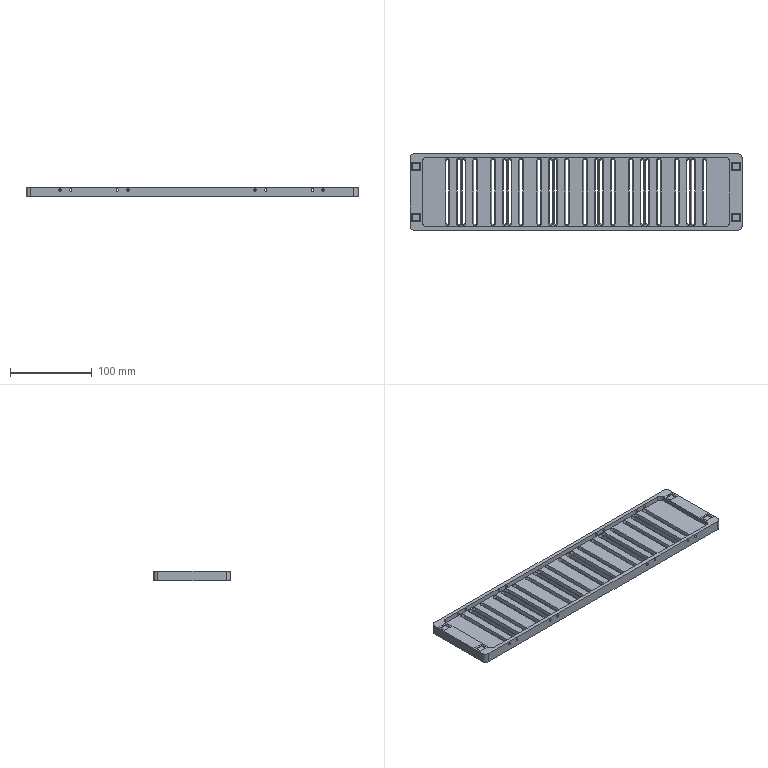Component | SolidWorks | MGL-PACK-01-00WeldedPlate1Assembly-1_MGL-PACK-01-01WeldPlate1-1 | 1 solid | 279 faces | box 405 x 93 x 12 mm | volume 214610 mm3 | plane 143 | cylinder 88 | cone 48 | commonest cylinder face diameters 3.5 x48 3 x32 10 x8
build123d program:
from build123d import *

# Parameters (mm, degrees)
SKETCH1_W             = 405
SKETCH1_H             = 93
BOSS_EXTRUDE1_DEPTH   = 12
CUT_EXTRUDE1_DEPTH    = 12
CUT_EXTRUDE4_DEPTH    = 12
LPATTERN1_COUNT       = 5
LPATTERN1_PITCH       = 56
CUT_EXTRUDE2_DEPTH    = 6
FILLET1_R             = 5
M3_TAPPED_HOLE1_D     = 3
M3_TAPPED_HOLE1_DEPTH = 120
M3_TAPPED_HOLE1_TIP   = 0.9013
SKETCH6_W             = 9
SKETCH6_H             = 8
CUT_EXTRUDE3_DEPTH    = 2
CHAMFER3_SIZE         = 1
CHAMFER4_SIZE         = 1
CHAMFER4_SIZE2        = 3.732


with BuildPart() as part:
    # Sketch1 → Boss-Extrude1 (new body)
    with BuildSketch(Plane.XY):
        Rectangle(SKETCH1_W, SKETCH1_H)
    extrude(amount=BOSS_EXTRUDE1_DEPTH)

    # Sketch2 → Cut-Extrude1 (cut)
    with BuildSketch(Plane.XY.offset(12)):
        with BuildLine():
            Line((-155.25, 38), (-155.25, -38))
            ThreePointArc((-155.25, -38), (-157, -39.75), (-158.75, -38))
            Line((-158.75, -38), (-158.75, 38))
            ThreePointArc((-158.75, 38), (-157, 39.75), (-155.25, 38))
        make_face()
        with BuildLine():
            Line((158.75, 38), (158.75, -38))
            ThreePointArc((158.75, -38), (157, -39.75), (155.25, -38))
            Line((155.25, -38), (155.25, 38))
            ThreePointArc((155.25, 38), (157, 39.75), (158.75, 38))
        make_face()
        with BuildLine():
            Line((-141.25, 38), (-141.25, -38))
            ThreePointArc((-141.25, -38), (-143, -39.75), (-144.75, -38))
            Line((-144.75, -38), (-144.75, 38))
            ThreePointArc((-144.75, 38), (-143, 39.75), (-141.25, 38))
        make_face()
        with BuildLine():
            Line((144.75, 38), (144.75, -38))
            ThreePointArc((144.75, -38), (143, -39.75), (141.25, -38))
            Line((141.25, -38), (141.25, 38))
            ThreePointArc((141.25, 38), (143, 39.75), (144.75, 38))
        make_face()
    extrude(amount=-CUT_EXTRUDE1_DEPTH, mode=Mode.SUBTRACT)

    # Sketch8 → Cut-Extrude4 (cut)
    with BuildSketch(Plane.XY.offset(12)):
        with BuildLine():
            Line((-135.25, 38), (-135.25, -38))
            ThreePointArc((-135.25, -38), (-137, -39.75), (-138.75, -38))
            Line((-138.75, -38), (-138.75, 38))
            ThreePointArc((-138.75, 38), (-137, 39.75), (-135.25, 38))
        make_face()
        with BuildLine():
            Line((-121.25, 38), (-121.25, -38))
            ThreePointArc((-121.25, -38), (-123, -39.75), (-124.75, -38))
            Line((-124.75, -38), (-124.75, 38))
            ThreePointArc((-124.75, 38), (-123, 39.75), (-121.25, 38))
        make_face()
        with BuildLine():
            Line((-99.25, 38), (-99.25, -38))
            ThreePointArc((-99.25, -38), (-101, -39.75), (-102.75, -38))
            Line((-102.75, -38), (-102.75, 38))
            ThreePointArc((-102.75, 38), (-101, 39.75), (-99.25, 38))
        make_face()
        with BuildLine():
            Line((-85.25, 38), (-85.25, -38))
            ThreePointArc((-85.25, -38), (-87, -39.75), (-88.75, -38))
            Line((-88.75, -38), (-88.75, 38))
            ThreePointArc((-88.75, 38), (-87, 39.75), (-85.25, 38))
        make_face()
    cut_extrude4 = extrude(amount=-CUT_EXTRUDE4_DEPTH, mode=Mode.SUBTRACT)

    # LPattern1: Cut-Extrude4 ×5
    with Locations(*[(i * LPATTERN1_PITCH, 0, 0) for i in range(1, LPATTERN1_COUNT)]):
        add(cut_extrude4, mode=Mode.SUBTRACT)

    # Sketch3 → Cut-Extrude2 (cut)
    with BuildSketch(Plane.XY.offset(12)):
        with BuildLine():
            Line((-182.5, 42), (182.5, 42))
            ThreePointArc((182.5, 42), (186.036, 40.536), (187.5, 37))
            Line((187.5, 37), (187.5, -37))
            ThreePointArc((187.5, -37), (186.036, -40.536), (182.5, -42))
            Line((182.5, -42), (-182.5, -42))
            ThreePointArc((-182.5, -42), (-186.036, -40.536), (-187.5, -37))
            Line((-187.5, -37), (-187.5, 37))
            ThreePointArc((-187.5, 37), (-186.036, 40.536), (-182.5, 42))
        make_face()
    extrude(amount=-CUT_EXTRUDE2_DEPTH, mode=Mode.SUBTRACT)

    # Fillet1
    fillet1_edges = [part.edges().sort_by_distance(p)[0] for p in [
        (-202.5, 46.5, 6),
        (202.5, 46.5, 6),
        (202.5, -46.5, 6),
        (-202.5, -46.5, 6),
    ]]
    fillet(fillet1_edges, radius=FILLET1_R)

    # M3 Tapped Hole1
    with Locations(Plane(origin=(0, 46.5, 0), x_dir=(1, 0, 0), z_dir=(0, 1, 0))):
        with Locations((-161.05, -8.5), (-148.05, -8.5), (146.95, -8.5), (159.95, -8.5), (-91.05, -8.5), (-78.05, -8.5), (76.95, -8.5), (89.95, -8.5)):
            Hole(M3_TAPPED_HOLE1_D / 2, depth=M3_TAPPED_HOLE1_DEPTH)
            with Locations((0, 0, -(M3_TAPPED_HOLE1_DEPTH + M3_TAPPED_HOLE1_TIP / 2))):  # 118° drill point
                Cone(0, M3_TAPPED_HOLE1_D / 2, M3_TAPPED_HOLE1_TIP, mode=Mode.SUBTRACT)

    # Sketch6 → Cut-Extrude3 (cut)
    with BuildSketch(Plane.XY.offset(12)):
        with Locations((195, 31)):
            Rectangle(SKETCH6_W, SKETCH6_H)
        with Locations((195, -31)):
            Rectangle(SKETCH6_W, SKETCH6_H)
        with Locations((-195, 31)):
            Rectangle(SKETCH6_W, SKETCH6_H)
        with Locations((-195, -31)):
            Rectangle(SKETCH6_W, SKETCH6_H)
    extrude(amount=-CUT_EXTRUDE3_DEPTH, mode=Mode.SUBTRACT)

    # Chamfer3
    chamfer3_edges = [part.edges().sort_by_distance(p)[0] for p in [
        (190.5, 31, 12),
        (195, 27, 12),
        (199.5, 31, 12),
        (195, 35, 12),
        (190.5, -31, 12),
        (195, -35, 12),
        (199.5, -31, 12),
        (195, -27, 12),
        (-199.5, 31, 12),
        (-195, 27, 12),
        (-190.5, 31, 12),
        (-195, 35, 12),
        (-199.5, -31, 12),
        (-195, -35, 12),
        (-190.5, -31, 12),
        (-195, -27, 12),
    ]]
    chamfer(chamfer3_edges, length=CHAMFER3_SIZE)

    # Chamfer4
    chamfer4_edges = [part.edges().sort_by_distance(p)[0] for p in [
        (137, 39.75, 6),
        (135.25, 0, 6),
        (137, -39.75, 6),
        (138.75, 0, 6),
        (87, 39.75, 6),
        (85.25, 0, 6),
        (87, -39.75, 6),
        (88.75, 0, 6),
        (101, 39.75, 6),
        (99.25, 0, 6),
        (101, -39.75, 6),
        (102.75, 0, 6),
        (123, 39.75, 6),
        (121.25, 0, 6),
        (123, -39.75, 6),
        (124.75, 0, 6),
        (81, 39.75, 6),
        (79.25, 0, 6),
        (81, -39.75, 6),
        (82.75, 0, 6),
        (31, 39.75, 6),
        (29.25, 0, 6),
        (31, -39.75, 6),
        (32.75, 0, 6),
        (45, 39.75, 6),
        (43.25, 0, 6),
        (45, -39.75, 6),
        (46.75, 0, 6),
        (67, 39.75, 6),
        (65.25, 0, 6),
        (67, -39.75, 6),
        (68.75, 0, 6),
        (25, 39.75, 6),
        (23.25, 0, 6),
        (25, -39.75, 6),
        (26.75, 0, 6),
        (-25, 39.75, 6),
        (-26.75, 0, 6),
        (-25, -39.75, 6),
        (-23.25, 0, 6),
        (-11, 39.75, 6),
        (-12.75, 0, 6),
        (-11, -39.75, 6),
        (-9.25, 0, 6),
        (11, 39.75, 6),
        (9.25, 0, 6),
        (11, -39.75, 6),
        (12.75, 0, 6),
        (-29.25, 0, 6),
        (-31, 39.75, 6),
        (-32.75, 0, 6),
        (-31, -39.75, 6),
        (-79.25, 0, 6),
        (-81, 39.75, 6),
        (-82.75, 0, 6),
        (-81, -39.75, 6),
        (-65.25, 0, 6),
        (-67, 39.75, 6),
        (-68.75, 0, 6),
        (-67, -39.75, 6),
        (-43.25, 0, 6),
        (-45, 39.75, 6),
        (-46.75, 0, 6),
        (-45, -39.75, 6),
        (-85.25, 0, 6),
        (-87, 39.75, 6),
        (-88.75, 0, 6),
        (-87, -39.75, 6),
        (-99.25, 0, 6),
        (-101, 39.75, 6),
        (-102.75, 0, 6),
        (-101, -39.75, 6),
        (-121.25, 0, 6),
        (-123, 39.75, 6),
        (-124.75, 0, 6),
        (-123, -39.75, 6),
        (-135.25, 0, 6),
        (-137, 39.75, 6),
        (-138.75, 0, 6),
        (-137, -39.75, 6),
        (144.75, 0, 6),
        (143, 39.75, 6),
        (141.25, 0, 6),
        (143, -39.75, 6),
        (-141.25, 0, 6),
        (-143, 39.75, 6),
        (-144.75, 0, 6),
        (-143, -39.75, 6),
        (158.75, 0, 6),
        (157, 39.75, 6),
        (155.25, 0, 6),
        (157, -39.75, 6),
        (-155.25, 0, 6),
        (-157, 39.75, 6),
        (-158.75, 0, 6),
        (-157, -39.75, 6),
    ]]
    chamfer4_side = [part.faces().sort_by_distance(p)[0] for p in [
        (0, 0, 6),
    ]]
    chamfer(chamfer4_edges, length=CHAMFER4_SIZE, length2=CHAMFER4_SIZE2, reference=chamfer4_side[0])


solid = part.part